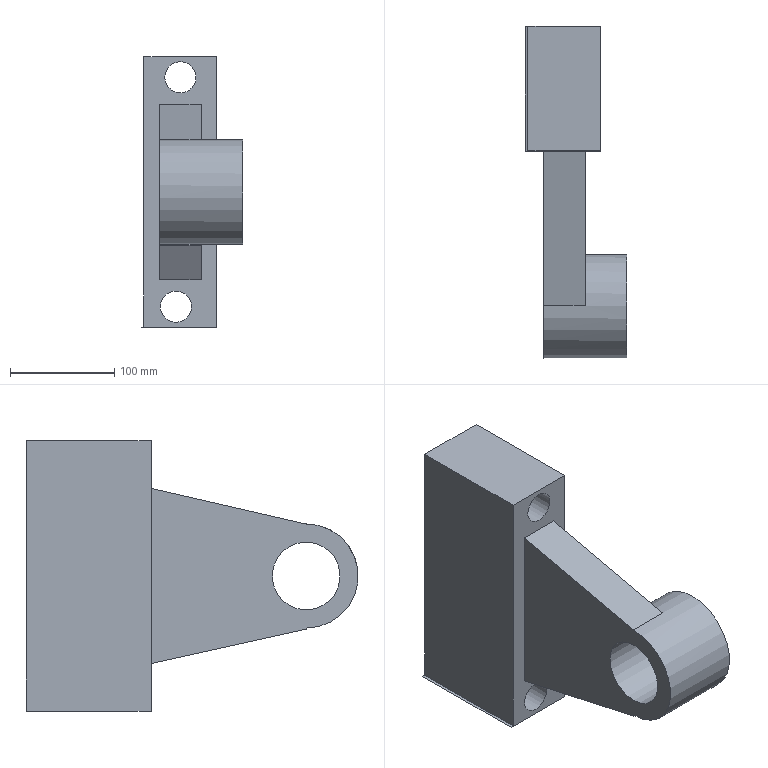Component | NX | BEARING_HOUSING_4 | 2 solids | 18 faces | volume 3022074 mm3 | plane 14 | cylinder 4 | commonest cylinder face diameters 30 x2 100 x1 65 x1